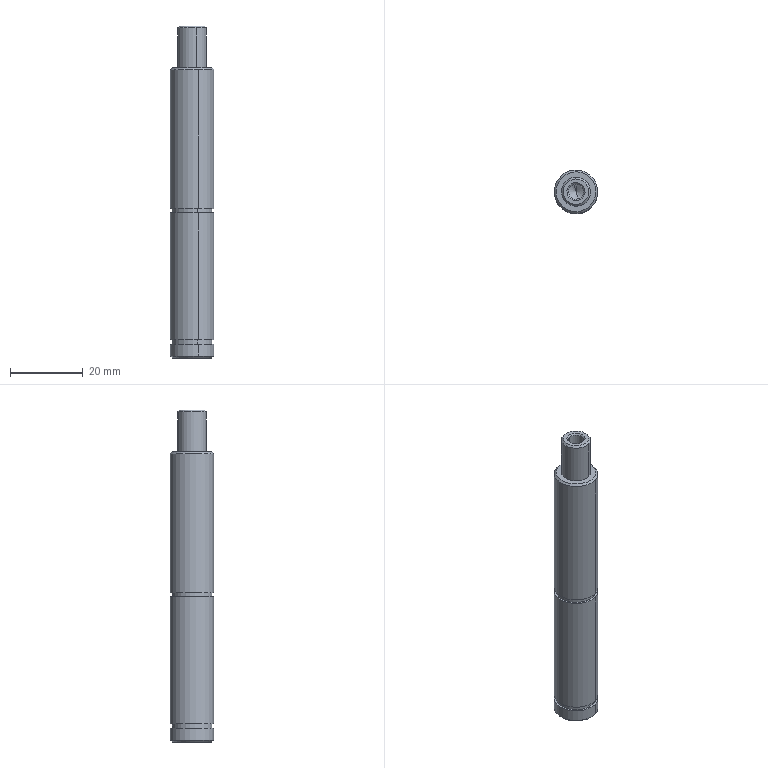Component | SolidWorks | GluePaperFeedingPressureRollerAssembly-1_YX-04-110GluePaperFeedingPressureRollerAxis-1 | 1 solid | 31 faces | box 12 x 12 x 91.5 mm | volume 9389 mm3 | cylinder 14 | cone 10 | plane 7 | commonest cylinder face diameters 12 x6 11 x4 8 x2 4.2 x2 | material Hard Chrome Rod
build123d program:
from build123d import *


with BuildPart() as part:
    # Sketch1 → Revolve1 (revolve)
    with BuildSketch(Plane.XY, mode=Mode.PRIVATE) as revolve1_sk:
        Polygon((12.6, 2.1), (13.862, 0), (91.5, 0), (91.5, 5.5), (91, 6), (87.7, 6), (87.7, 5.5), (86.5, 5.5), (86.5, 6), (51.5, 6), (51.5, 5.5), (50.3, 5.5), (50.3, 6), (12, 6), (11.5, 5.5), (11.5, 4), (0.5, 4), (0, 3.5), (0, 2.5), (0.4, 2.1), align=None)
    revolve(revolve1_sk.sketch.rotate(Axis((0, 0, 0), (1, 0, 0)), 270), axis=Axis((0, 0, 0), (1, 0, 0)))


solid = part.part

# Placed as in the assembly
solid = solid.moved(Location((-23.397, 0.262, 205.5), (0, 90, 0)))
STEP:
#1=CARTESIAN_POINT('',(-0.8978,-0.069,8.075));
#2=VERTEX_POINT('',#1);
#3=CARTESIAN_POINT('',(-0.9445,0.08963,8.075));
#4=VERTEX_POINT('',#3);
#5=CARTESIAN_POINT('',(-0.9212,0.01031,8.075));
#6=DIRECTION('',(-0.,0.,-1.));
#7=DIRECTION('',(-0.2824,0.9593,0.));
#8=AXIS2_PLACEMENT_3D('',#5,#6,#7);
#9=CIRCLE('',#8,0.08268);
#10=EDGE_CURVE('',#2,#4,#9,.T.);
#11=ORIENTED_EDGE('',*,*,#10,.T.);
#12=CARTESIAN_POINT('',(-0.9489,0.1047,8.091));
#13=VERTEX_POINT('',#12);
#14=CARTESIAN_POINT('',(-0.9489,0.1047,8.091));
#15=DIRECTION('',(-0.1997,0.6783,0.7071));
#16=VECTOR('',#15,39.37);
#17=LINE('',#14,#16);
#18=EDGE_CURVE('',#4,#13,#17,.T.);
#19=ORIENTED_EDGE('',*,*,#18,.T.);
#20=CARTESIAN_POINT('',(-0.8934,-0.0841,8.091));
#21=VERTEX_POINT('',#20);
#22=CARTESIAN_POINT('',(-0.9212,0.01031,8.091));
#23=DIRECTION('',(-0.,0.,-1.));
#24=DIRECTION('',(-0.2824,0.9593,0.));
#25=AXIS2_PLACEMENT_3D('',#22,#23,#24);
#26=CIRCLE('',#25,0.09843);
#27=EDGE_CURVE('',#21,#13,#26,.T.);
#28=ORIENTED_EDGE('',*,*,#27,.F.);
#29=CARTESIAN_POINT('',(-0.8934,-0.0841,8.091));
#30=DIRECTION('',(0.1997,-0.6783,0.7071));
#31=VECTOR('',#30,39.37);
#32=LINE('',#29,#31);
#33=EDGE_CURVE('',#2,#21,#32,.T.);
#34=ORIENTED_EDGE('',*,*,#33,.F.);
#35=EDGE_LOOP('',(#11,#19,#28,#34));
#36=FACE_OUTER_BOUND('',#35,.T.);
#37=CARTESIAN_POINT('',(-0.9212,0.01031,8.091));
#38=DIRECTION('',(0.,-0.,1.));
#39=DIRECTION('',(0.2824,-0.9593,0.));
#40=AXIS2_PLACEMENT_3D('',#37,#38,#39);
#41=CONICAL_SURFACE('',#40,0.09843,0.7854);
#42=ADVANCED_FACE('',(#36),#41,.F.);
#43=CARTESIAN_POINT('',(-0.9601,0.1425,8.091));
#44=VERTEX_POINT('',#43);
#45=CARTESIAN_POINT('',(-0.8822,-0.1219,8.091));
#46=VERTEX_POINT('',#45);
#47=CARTESIAN_POINT('',(-0.9212,0.01031,8.091));
#48=DIRECTION('',(-0.,0.,-1.));
#49=DIRECTION('',(-0.2824,0.9593,0.));
#50=AXIS2_PLACEMENT_3D('',#47,#48,#49);
#51=CIRCLE('',#50,0.1378);
#52=EDGE_CURVE('',#44,#46,#51,.T.);
#53=ORIENTED_EDGE('',*,*,#52,.T.);
#54=CARTESIAN_POINT('',(-0.8767,-0.1408,8.071));
#55=VERTEX_POINT('',#54);
#56=CARTESIAN_POINT('',(-0.8767,-0.1408,8.071));
#57=DIRECTION('',(0.1997,-0.6783,-0.7071));
#58=VECTOR('',#57,39.37);
#59=LINE('',#56,#58);
#60=EDGE_CURVE('',#46,#55,#59,.T.);
#61=ORIENTED_EDGE('',*,*,#60,.T.);
#62=CARTESIAN_POINT('',(-0.9656,0.1614,8.071));
#63=VERTEX_POINT('',#62);
#64=CARTESIAN_POINT('',(-0.9212,0.01031,8.071));
#65=DIRECTION('',(-0.,0.,-1.));
#66=DIRECTION('',(-0.2824,0.9593,0.));
#67=AXIS2_PLACEMENT_3D('',#64,#65,#66);
#68=CIRCLE('',#67,0.1575);
#69=EDGE_CURVE('',#63,#55,#68,.T.);
#70=ORIENTED_EDGE('',*,*,#69,.F.);
#71=CARTESIAN_POINT('',(-0.9656,0.1614,8.071));
#72=DIRECTION('',(-0.1997,0.6783,-0.7071));
#73=VECTOR('',#72,39.37);
#74=LINE('',#71,#73);
#75=EDGE_CURVE('',#44,#63,#74,.T.);
#76=ORIENTED_EDGE('',*,*,#75,.F.);
#77=EDGE_LOOP('',(#53,#61,#70,#76));
#78=FACE_OUTER_BOUND('',#77,.T.);
#79=CARTESIAN_POINT('',(-0.9212,0.01031,8.071));
#80=DIRECTION('',(-0.,0.,-1.));
#81=DIRECTION('',(-0.2824,0.9593,0.));
#82=AXIS2_PLACEMENT_3D('',#79,#80,#81);
#83=CONICAL_SURFACE('',#82,0.1575,0.7854);
#84=ADVANCED_FACE('',(#78),#83,.T.);
#85=ORIENTED_EDGE('',*,*,#69,.T.);
#86=CARTESIAN_POINT('',(-0.8767,-0.1408,7.638));
#87=VERTEX_POINT('',#86);
#88=CARTESIAN_POINT('',(-0.8767,-0.1408,8.091));
#89=DIRECTION('',(-0.,0.,-1.));
#90=VECTOR('',#89,39.37);
#91=LINE('',#88,#90);
#92=EDGE_CURVE('',#55,#87,#91,.T.);
#93=ORIENTED_EDGE('',*,*,#92,.T.);
#94=CARTESIAN_POINT('',(-0.9656,0.1614,7.638));
#95=VERTEX_POINT('',#94);
#96=CARTESIAN_POINT('',(-0.9212,0.01031,7.638));
#97=DIRECTION('',(-0.,0.,-1.));
#98=DIRECTION('',(-0.2824,0.9593,0.));
#99=AXIS2_PLACEMENT_3D('',#96,#97,#98);
#100=CIRCLE('',#99,0.1575);
#101=EDGE_CURVE('',#95,#87,#100,.T.);
#102=ORIENTED_EDGE('',*,*,#101,.F.);
#103=CARTESIAN_POINT('',(-0.9656,0.1614,8.091));
#104=DIRECTION('',(-0.,0.,-1.));
#105=VECTOR('',#104,39.37);
#106=LINE('',#103,#105);
#107=EDGE_CURVE('',#63,#95,#106,.T.);
#108=ORIENTED_EDGE('',*,*,#107,.F.);
#109=EDGE_LOOP('',(#85,#93,#102,#108));
#110=FACE_OUTER_BOUND('',#109,.T.);
#111=CARTESIAN_POINT('',(-0.9212,0.01031,8.091));
#112=DIRECTION('',(-0.,0.,-1.));
#113=DIRECTION('',(-0.2824,0.9593,0.));
#114=AXIS2_PLACEMENT_3D('',#111,#112,#113);
#115=CYLINDRICAL_SURFACE('',#114,0.1575);
#116=ADVANCED_FACE('',(#110),#115,.T.);
#117=CARTESIAN_POINT('',(-0.9823,0.218,7.638));
#118=VERTEX_POINT('',#117);
#119=CARTESIAN_POINT('',(-0.86,-0.1974,7.638));
#120=VERTEX_POINT('',#119);
#121=CARTESIAN_POINT('',(-0.9212,0.01031,7.638));
#122=DIRECTION('',(-0.,0.,-1.));
#123=DIRECTION('',(-0.2824,0.9593,0.));
#124=AXIS2_PLACEMENT_3D('',#121,#122,#123);
#125=CIRCLE('',#124,0.2165);
#126=EDGE_CURVE('',#118,#120,#125,.T.);
#127=ORIENTED_EDGE('',*,*,#126,.T.);
#128=CARTESIAN_POINT('',(-0.8544,-0.2163,7.618));
#129=VERTEX_POINT('',#128);
#130=CARTESIAN_POINT('',(-0.8544,-0.2163,7.618));
#131=DIRECTION('',(0.1997,-0.6783,-0.7071));
#132=VECTOR('',#131,39.37);
#133=LINE('',#130,#132);
#134=EDGE_CURVE('',#120,#129,#133,.T.);
#135=ORIENTED_EDGE('',*,*,#134,.T.);
#136=CARTESIAN_POINT('',(-0.9879,0.2369,7.618));
#137=VERTEX_POINT('',#136);
#138=CARTESIAN_POINT('',(-0.9212,0.01031,7.618));
#139=DIRECTION('',(-0.,0.,-1.));
#140=DIRECTION('',(-0.2824,0.9593,0.));
#141=AXIS2_PLACEMENT_3D('',#138,#139,#140);
#142=CIRCLE('',#141,0.2362);
#143=EDGE_CURVE('',#137,#129,#142,.T.);
#144=ORIENTED_EDGE('',*,*,#143,.F.);
#145=CARTESIAN_POINT('',(-0.9879,0.2369,7.618));
#146=DIRECTION('',(-0.1997,0.6783,-0.7071));
#147=VECTOR('',#146,39.37);
#148=LINE('',#145,#147);
#149=EDGE_CURVE('',#118,#137,#148,.T.);
#150=ORIENTED_EDGE('',*,*,#149,.F.);
#151=EDGE_LOOP('',(#127,#135,#144,#150));
#152=FACE_OUTER_BOUND('',#151,.T.);
#153=CARTESIAN_POINT('',(-0.9212,0.01031,7.618));
#154=DIRECTION('',(-0.,0.,-1.));
#155=DIRECTION('',(-0.2824,0.9593,0.));
#156=AXIS2_PLACEMENT_3D('',#153,#154,#155);
#157=CONICAL_SURFACE('',#156,0.2362,0.7854);
#158=ADVANCED_FACE('',(#152),#157,.T.);
#159=ORIENTED_EDGE('',*,*,#143,.T.);
#160=CARTESIAN_POINT('',(-0.8544,-0.2163,6.11));
#161=VERTEX_POINT('',#160);
#162=CARTESIAN_POINT('',(-0.8544,-0.2163,8.091));
#163=DIRECTION('',(-0.,0.,-1.));
#164=VECTOR('',#163,39.37);
#165=LINE('',#162,#164);
#166=EDGE_CURVE('',#129,#161,#165,.T.);
#167=ORIENTED_EDGE('',*,*,#166,.T.);
#168=CARTESIAN_POINT('',(-0.9879,0.2369,6.11));
#169=VERTEX_POINT('',#168);
#170=CARTESIAN_POINT('',(-0.9212,0.01031,6.11));
#171=DIRECTION('',(-0.,0.,-1.));
#172=DIRECTION('',(-0.2824,0.9593,0.));
#173=AXIS2_PLACEMENT_3D('',#170,#171,#172);
#174=CIRCLE('',#173,0.2362);
#175=EDGE_CURVE('',#169,#161,#174,.T.);
#176=ORIENTED_EDGE('',*,*,#175,.F.);
#177=CARTESIAN_POINT('',(-0.9879,0.2369,8.091));
#178=DIRECTION('',(-0.,0.,-1.));
#179=VECTOR('',#178,39.37);
#180=LINE('',#177,#179);
#181=EDGE_CURVE('',#137,#169,#180,.T.);
#182=ORIENTED_EDGE('',*,*,#181,.F.);
#183=EDGE_LOOP('',(#159,#167,#176,#182));
#184=FACE_OUTER_BOUND('',#183,.T.);
#185=CARTESIAN_POINT('',(-0.9212,0.01031,8.091));
#186=DIRECTION('',(-0.,0.,-1.));
#187=DIRECTION('',(-0.2824,0.9593,0.));
#188=AXIS2_PLACEMENT_3D('',#185,#186,#187);
#189=CYLINDRICAL_SURFACE('',#188,0.2362);
#190=ADVANCED_FACE('',(#184),#189,.T.);
#191=CARTESIAN_POINT('',(-0.9823,0.218,6.11));
#192=VERTEX_POINT('',#191);
#193=CARTESIAN_POINT('',(-0.86,-0.1974,6.11));
#194=VERTEX_POINT('',#193);
#195=CARTESIAN_POINT('',(-0.9212,0.01031,6.11));
#196=DIRECTION('',(-0.,0.,-1.));
#197=DIRECTION('',(-0.2824,0.9593,0.));
#198=AXIS2_PLACEMENT_3D('',#195,#196,#197);
#199=CIRCLE('',#198,0.2165);
#200=EDGE_CURVE('',#192,#194,#199,.T.);
#201=ORIENTED_EDGE('',*,*,#200,.T.);
#202=CARTESIAN_POINT('',(-0.86,-0.1974,6.063));
#203=VERTEX_POINT('',#202);
#204=CARTESIAN_POINT('',(-0.86,-0.1974,8.091));
#205=DIRECTION('',(-0.,0.,-1.));
#206=VECTOR('',#205,39.37);
#207=LINE('',#204,#206);
#208=EDGE_CURVE('',#194,#203,#207,.T.);
#209=ORIENTED_EDGE('',*,*,#208,.T.);
#210=CARTESIAN_POINT('',(-0.9823,0.218,6.063));
#211=VERTEX_POINT('',#210);
#212=CARTESIAN_POINT('',(-0.9212,0.01031,6.063));
#213=DIRECTION('',(-0.,0.,-1.));
#214=DIRECTION('',(-0.2824,0.9593,0.));
#215=AXIS2_PLACEMENT_3D('',#212,#213,#214);
#216=CIRCLE('',#215,0.2165);
#217=EDGE_CURVE('',#211,#203,#216,.T.);
#218=ORIENTED_EDGE('',*,*,#217,.F.);
#219=CARTESIAN_POINT('',(-0.9823,0.218,8.091));
#220=DIRECTION('',(-0.,0.,-1.));
#221=VECTOR('',#220,39.37);
#222=LINE('',#219,#221);
#223=EDGE_CURVE('',#192,#211,#222,.T.);
#224=ORIENTED_EDGE('',*,*,#223,.F.);
#225=EDGE_LOOP('',(#201,#209,#218,#224));
#226=FACE_OUTER_BOUND('',#225,.T.);
#227=CARTESIAN_POINT('',(-0.9212,0.01031,8.091));
#228=DIRECTION('',(-0.,0.,-1.));
#229=DIRECTION('',(-0.2824,0.9593,0.));
#230=AXIS2_PLACEMENT_3D('',#227,#228,#229);
#231=CYLINDRICAL_SURFACE('',#230,0.2165);
#232=ADVANCED_FACE('',(#226),#231,.T.);
#233=CARTESIAN_POINT('',(-0.9879,0.2369,6.063));
#234=VERTEX_POINT('',#233);
#235=CARTESIAN_POINT('',(-0.8544,-0.2163,6.063));
#236=VERTEX_POINT('',#235);
#237=CARTESIAN_POINT('',(-0.9212,0.01031,6.063));
#238=DIRECTION('',(-0.,0.,-1.));
#239=DIRECTION('',(-0.2824,0.9593,0.));
#240=AXIS2_PLACEMENT_3D('',#237,#238,#239);
#241=CIRCLE('',#240,0.2362);
#242=EDGE_CURVE('',#234,#236,#241,.T.);
#243=ORIENTED_EDGE('',*,*,#242,.T.);
#244=CARTESIAN_POINT('',(-0.8544,-0.2163,4.685));
#245=VERTEX_POINT('',#244);
#246=CARTESIAN_POINT('',(-0.8544,-0.2163,8.091));
#247=DIRECTION('',(-0.,0.,-1.));
#248=VECTOR('',#247,39.37);
#249=LINE('',#246,#248);
#250=EDGE_CURVE('',#236,#245,#249,.T.);
#251=ORIENTED_EDGE('',*,*,#250,.T.);
#252=CARTESIAN_POINT('',(-0.9879,0.2369,4.685));
#253=VERTEX_POINT('',#252);
#254=CARTESIAN_POINT('',(-0.9212,0.01031,4.685));
#255=DIRECTION('',(-0.,0.,-1.));
#256=DIRECTION('',(-0.2824,0.9593,0.));
#257=AXIS2_PLACEMENT_3D('',#254,#255,#256);
#258=CIRCLE('',#257,0.2362);
#259=EDGE_CURVE('',#253,#245,#258,.T.);
#260=ORIENTED_EDGE('',*,*,#259,.F.);
#261=CARTESIAN_POINT('',(-0.9879,0.2369,8.091));
#262=DIRECTION('',(-0.,0.,-1.));
#263=VECTOR('',#262,39.37);
#264=LINE('',#261,#263);
#265=EDGE_CURVE('',#234,#253,#264,.T.);
#266=ORIENTED_EDGE('',*,*,#265,.F.);
#267=EDGE_LOOP('',(#243,#251,#260,#266));
#268=FACE_OUTER_BOUND('',#267,.T.);
#269=CARTESIAN_POINT('',(-0.9212,0.01031,8.091));
#270=DIRECTION('',(-0.,0.,-1.));
#271=DIRECTION('',(-0.2824,0.9593,0.));
#272=AXIS2_PLACEMENT_3D('',#269,#270,#271);
#273=CYLINDRICAL_SURFACE('',#272,0.2362);
#274=ADVANCED_FACE('',(#268),#273,.T.);
#275=CARTESIAN_POINT('',(-0.9823,0.218,4.685));
#276=VERTEX_POINT('',#275);
#277=CARTESIAN_POINT('',(-0.86,-0.1974,4.685));
#278=VERTEX_POINT('',#277);
#279=CARTESIAN_POINT('',(-0.9212,0.01031,4.685));
#280=DIRECTION('',(-0.,0.,-1.));
#281=DIRECTION('',(-0.2824,0.9593,0.));
#282=AXIS2_PLACEMENT_3D('',#279,#280,#281);
#283=CIRCLE('',#282,0.2165);
#284=EDGE_CURVE('',#276,#278,#283,.T.);
#285=ORIENTED_EDGE('',*,*,#284,.T.);
#286=CARTESIAN_POINT('',(-0.86,-0.1974,4.638));
#287=VERTEX_POINT('',#286);
#288=CARTESIAN_POINT('',(-0.86,-0.1974,8.091));
#289=DIRECTION('',(-0.,0.,-1.));
#290=VECTOR('',#289,39.37);
#291=LINE('',#288,#290);
#292=EDGE_CURVE('',#278,#287,#291,.T.);
#293=ORIENTED_EDGE('',*,*,#292,.T.);
#294=CARTESIAN_POINT('',(-0.9823,0.218,4.638));
#295=VERTEX_POINT('',#294);
#296=CARTESIAN_POINT('',(-0.9212,0.01031,4.638));
#297=DIRECTION('',(-0.,0.,-1.));
#298=DIRECTION('',(-0.2824,0.9593,0.));
#299=AXIS2_PLACEMENT_3D('',#296,#297,#298);
#300=CIRCLE('',#299,0.2165);
#301=EDGE_CURVE('',#295,#287,#300,.T.);
#302=ORIENTED_EDGE('',*,*,#301,.F.);
#303=CARTESIAN_POINT('',(-0.9823,0.218,8.091));
#304=DIRECTION('',(-0.,0.,-1.));
#305=VECTOR('',#304,39.37);
#306=LINE('',#303,#305);
#307=EDGE_CURVE('',#276,#295,#306,.T.);
#308=ORIENTED_EDGE('',*,*,#307,.F.);
#309=EDGE_LOOP('',(#285,#293,#302,#308));
#310=FACE_OUTER_BOUND('',#309,.T.);
#311=CARTESIAN_POINT('',(-0.9212,0.01031,8.091));
#312=DIRECTION('',(-0.,0.,-1.));
#313=DIRECTION('',(-0.2824,0.9593,0.));
#314=AXIS2_PLACEMENT_3D('',#311,#312,#313);
#315=CYLINDRICAL_SURFACE('',#314,0.2165);
#316=ADVANCED_FACE('',(#310),#315,.T.);
#317=CARTESIAN_POINT('',(-0.9879,0.2369,4.638));
#318=VERTEX_POINT('',#317);
#319=CARTESIAN_POINT('',(-0.8544,-0.2163,4.638));
#320=VERTEX_POINT('',#319);
#321=CARTESIAN_POINT('',(-0.9212,0.01031,4.638));
#322=DIRECTION('',(-0.,0.,-1.));
#323=DIRECTION('',(-0.2824,0.9593,0.));
#324=AXIS2_PLACEMENT_3D('',#321,#322,#323);
#325=CIRCLE('',#324,0.2362);
#326=EDGE_CURVE('',#318,#320,#325,.T.);
#327=ORIENTED_EDGE('',*,*,#326,.T.);
#328=CARTESIAN_POINT('',(-0.8544,-0.2163,4.508));
#329=VERTEX_POINT('',#328);
#330=CARTESIAN_POINT('',(-0.8544,-0.2163,8.091));
#331=DIRECTION('',(-0.,0.,-1.));
#332=VECTOR('',#331,39.37);
#333=LINE('',#330,#332);
#334=EDGE_CURVE('',#320,#329,#333,.T.);
#335=ORIENTED_EDGE('',*,*,#334,.T.);
#336=CARTESIAN_POINT('',(-0.9879,0.2369,4.508));
#337=VERTEX_POINT('',#336);
#338=CARTESIAN_POINT('',(-0.9212,0.01031,4.508));
#339=DIRECTION('',(-0.,0.,-1.));
#340=DIRECTION('',(-0.2824,0.9593,0.));
#341=AXIS2_PLACEMENT_3D('',#338,#339,#340);
#342=CIRCLE('',#341,0.2362);
#343=EDGE_CURVE('',#337,#329,#342,.T.);
#344=ORIENTED_EDGE('',*,*,#343,.F.);
#345=CARTESIAN_POINT('',(-0.9879,0.2369,8.091));
#346=DIRECTION('',(-0.,0.,-1.));
#347=VECTOR('',#346,39.37);
#348=LINE('',#345,#347);
#349=EDGE_CURVE('',#318,#337,#348,.T.);
#350=ORIENTED_EDGE('',*,*,#349,.F.);
#351=EDGE_LOOP('',(#327,#335,#344,#350));
#352=FACE_OUTER_BOUND('',#351,.T.);
#353=CARTESIAN_POINT('',(-0.9212,0.01031,8.091));
#354=DIRECTION('',(-0.,0.,-1.));
#355=DIRECTION('',(-0.2824,0.9593,0.));
#356=AXIS2_PLACEMENT_3D('',#353,#354,#355);
#357=CYLINDRICAL_SURFACE('',#356,0.2362);
#358=ADVANCED_FACE('',(#352),#357,.T.);
#359=CARTESIAN_POINT('',(-0.9823,0.218,4.488));
#360=VERTEX_POINT('',#359);
#361=CARTESIAN_POINT('',(-0.86,-0.1974,4.488));
#362=VERTEX_POINT('',#361);
#363=CARTESIAN_POINT('',(-0.9212,0.01031,4.488));
#364=DIRECTION('',(-0.,0.,-1.));
#365=DIRECTION('',(-0.2824,0.9593,0.));
#366=AXIS2_PLACEMENT_3D('',#363,#364,#365);
#367=CIRCLE('',#366,0.2165);
#368=EDGE_CURVE('',#360,#362,#367,.T.);
#369=ORIENTED_EDGE('',*,*,#368,.F.);
#370=CARTESIAN_POINT('',(-0.9823,0.218,4.488));
#371=DIRECTION('',(-0.1997,0.6783,0.7071));
#372=VECTOR('',#371,39.37);
#373=LINE('',#370,#372);
#374=EDGE_CURVE('',#360,#337,#373,.T.);
#375=ORIENTED_EDGE('',*,*,#374,.T.);
#376=ORIENTED_EDGE('',*,*,#343,.T.);
#377=CARTESIAN_POINT('',(-0.86,-0.1974,4.488));
#378=DIRECTION('',(0.1997,-0.6783,0.7071));
#379=VECTOR('',#378,39.37);
#380=LINE('',#377,#379);
#381=EDGE_CURVE('',#362,#329,#380,.T.);
#382=ORIENTED_EDGE('',*,*,#381,.F.);
#383=EDGE_LOOP('',(#369,#375,#376,#382));
#384=FACE_OUTER_BOUND('',#383,.T.);
#385=CARTESIAN_POINT('',(-0.9212,0.01031,4.488));
#386=DIRECTION('',(0.,-0.,1.));
#387=DIRECTION('',(0.2824,-0.9593,0.));
#388=AXIS2_PLACEMENT_3D('',#385,#386,#387);
#389=CONICAL_SURFACE('',#388,0.2165,0.7854);
#390=ADVANCED_FACE('',(#384),#389,.T.);
#391=CARTESIAN_POINT('',(-0.9212,0.01031,7.545));
#392=VERTEX_POINT('',#391);
#393=CARTESIAN_POINT('',(-0.8978,-0.069,7.594));
#394=VERTEX_POINT('',#393);
#395=CARTESIAN_POINT('',(-0.8978,-0.069,7.594));
#396=DIRECTION('',(0.2421,-0.8223,0.515));
#397=VECTOR('',#396,39.37);
#398=LINE('',#395,#397);
#399=EDGE_CURVE('',#392,#394,#398,.T.);
#400=ORIENTED_EDGE('',*,*,#399,.F.);
#401=CARTESIAN_POINT('',(-0.9445,0.08963,7.594));
#402=VERTEX_POINT('',#401);
#403=CARTESIAN_POINT('',(-0.9445,0.08963,7.594));
#404=DIRECTION('',(-0.2421,0.8223,0.515));
#405=VECTOR('',#404,39.37);
#406=LINE('',#403,#405);
#407=EDGE_CURVE('',#392,#402,#406,.T.);
#408=ORIENTED_EDGE('',*,*,#407,.T.);
#409=CARTESIAN_POINT('',(-0.9212,0.01031,7.594));
#410=DIRECTION('',(-0.,0.,-1.));
#411=DIRECTION('',(-0.2824,0.9593,0.));
#412=AXIS2_PLACEMENT_3D('',#409,#410,#411);
#413=CIRCLE('',#412,0.08268);
#414=EDGE_CURVE('',#394,#402,#413,.T.);
#415=ORIENTED_EDGE('',*,*,#414,.F.);
#416=EDGE_LOOP('',(#400,#408,#415));
#417=FACE_OUTER_BOUND('',#416,.T.);
#418=CARTESIAN_POINT('',(-0.9212,0.01031,7.594));
#419=DIRECTION('',(0.,-0.,1.));
#420=DIRECTION('',(0.2824,-0.9593,0.));
#421=AXIS2_PLACEMENT_3D('',#418,#419,#420);
#422=CONICAL_SURFACE('',#421,0.08268,1.03);
#423=ADVANCED_FACE('',(#417),#422,.F.);
#424=ORIENTED_EDGE('',*,*,#10,.F.);
#425=CARTESIAN_POINT('',(-0.8978,-0.069,8.091));
#426=DIRECTION('',(-0.,0.,-1.));
#427=VECTOR('',#426,39.37);
#428=LINE('',#425,#427);
#429=EDGE_CURVE('',#2,#394,#428,.T.);
#430=ORIENTED_EDGE('',*,*,#429,.T.);
#431=ORIENTED_EDGE('',*,*,#414,.T.);
#432=CARTESIAN_POINT('',(-0.9445,0.08963,8.091));
#433=DIRECTION('',(-0.,0.,-1.));
#434=VECTOR('',#433,39.37);
#435=LINE('',#432,#434);
#436=EDGE_CURVE('',#4,#402,#435,.T.);
#437=ORIENTED_EDGE('',*,*,#436,.F.);
#438=EDGE_LOOP('',(#424,#430,#431,#437));
#439=FACE_OUTER_BOUND('',#438,.T.);
#440=CARTESIAN_POINT('',(-0.9212,0.01031,8.091));
#441=DIRECTION('',(-0.,0.,-1.));
#442=DIRECTION('',(-0.2824,0.9593,0.));
#443=AXIS2_PLACEMENT_3D('',#440,#441,#442);
#444=CYLINDRICAL_SURFACE('',#443,0.08268);
#445=ADVANCED_FACE('',(#439),#444,.F.);
#446=ORIENTED_EDGE('',*,*,#429,.F.);
#447=CARTESIAN_POINT('',(-0.9212,0.01031,8.075));
#448=DIRECTION('',(-0.,0.,-1.));
#449=DIRECTION('',(-0.2824,0.9593,0.));
#450=AXIS2_PLACEMENT_3D('',#447,#448,#449);
#451=CIRCLE('',#450,0.08268);
#452=EDGE_CURVE('',#4,#2,#451,.T.);
#453=ORIENTED_EDGE('',*,*,#452,.F.);
#454=ORIENTED_EDGE('',*,*,#436,.T.);
#455=CARTESIAN_POINT('',(-0.9212,0.01031,7.594));
#456=DIRECTION('',(-0.,0.,-1.));
#457=DIRECTION('',(-0.2824,0.9593,0.));
#458=AXIS2_PLACEMENT_3D('',#455,#456,#457);
#459=CIRCLE('',#458,0.08268);
#460=EDGE_CURVE('',#402,#394,#459,.T.);
#461=ORIENTED_EDGE('',*,*,#460,.T.);
#462=EDGE_LOOP('',(#446,#453,#454,#461));
#463=FACE_OUTER_BOUND('',#462,.T.);
#464=CARTESIAN_POINT('',(-0.9212,0.01031,8.091));
#465=DIRECTION('',(-0.,0.,-1.));
#466=DIRECTION('',(-0.2824,0.9593,0.));
#467=AXIS2_PLACEMENT_3D('',#464,#465,#466);
#468=CYLINDRICAL_SURFACE('',#467,0.08268);
#469=ADVANCED_FACE('',(#463),#468,.F.);
#470=ORIENTED_EDGE('',*,*,#407,.F.);
#471=ORIENTED_EDGE('',*,*,#399,.T.);
#472=ORIENTED_EDGE('',*,*,#460,.F.);
#473=EDGE_LOOP('',(#470,#471,#472));
#474=FACE_OUTER_BOUND('',#473,.T.);
#475=CARTESIAN_POINT('',(-0.9212,0.01031,7.594));
#476=DIRECTION('',(0.,-0.,1.));
#477=DIRECTION('',(0.2824,-0.9593,0.));
#478=AXIS2_PLACEMENT_3D('',#475,#476,#477);
#479=CONICAL_SURFACE('',#478,0.08268,1.03);
#480=ADVANCED_FACE('',(#474),#479,.F.);
#481=CARTESIAN_POINT('',(-0.9212,0.01031,4.488));
#482=DIRECTION('',(-0.,0.,-1.));
#483=DIRECTION('',(-0.2824,0.9593,0.));
#484=AXIS2_PLACEMENT_3D('',#481,#482,#483);
#485=CIRCLE('',#484,0.2165);
#486=EDGE_CURVE('',#362,#360,#485,.T.);
#487=ORIENTED_EDGE('',*,*,#486,.T.);
#488=ORIENTED_EDGE('',*,*,#368,.T.);
#489=EDGE_LOOP('',(#487,#488));
#490=FACE_OUTER_BOUND('',#489,.T.);
#491=CARTESIAN_POINT('',(-0.9212,0.01031,4.488));
#492=DIRECTION('',(-0.,0.,-1.));
#493=DIRECTION('',(-0.2824,0.9593,0.));
#494=AXIS2_PLACEMENT_3D('',#491,#492,#493);
#495=PLANE('',#494);
#496=ADVANCED_FACE('',(#490),#495,.T.);
#497=ORIENTED_EDGE('',*,*,#374,.F.);
#498=ORIENTED_EDGE('',*,*,#486,.F.);
#499=ORIENTED_EDGE('',*,*,#381,.T.);
#500=CARTESIAN_POINT('',(-0.9212,0.01031,4.508));
#501=DIRECTION('',(-0.,0.,-1.));
#502=DIRECTION('',(-0.2824,0.9593,0.));
#503=AXIS2_PLACEMENT_3D('',#500,#501,#502);
#504=CIRCLE('',#503,0.2362);
#505=EDGE_CURVE('',#329,#337,#504,.T.);
#506=ORIENTED_EDGE('',*,*,#505,.T.);
#507=EDGE_LOOP('',(#497,#498,#499,#506));
#508=FACE_OUTER_BOUND('',#507,.T.);
#509=CARTESIAN_POINT('',(-0.9212,0.01031,4.488));
#510=DIRECTION('',(0.,-0.,1.));
#511=DIRECTION('',(0.2824,-0.9593,0.));
#512=AXIS2_PLACEMENT_3D('',#509,#510,#511);
#513=CONICAL_SURFACE('',#512,0.2165,0.7854);
#514=ADVANCED_FACE('',(#508),#513,.T.);
#515=ORIENTED_EDGE('',*,*,#334,.F.);
#516=CARTESIAN_POINT('',(-0.9212,0.01031,4.638));
#517=DIRECTION('',(-0.,0.,-1.));
#518=DIRECTION('',(-0.2824,0.9593,0.));
#519=AXIS2_PLACEMENT_3D('',#516,#517,#518);
#520=CIRCLE('',#519,0.2362);
#521=EDGE_CURVE('',#320,#318,#520,.T.);
#522=ORIENTED_EDGE('',*,*,#521,.T.);
#523=ORIENTED_EDGE('',*,*,#349,.T.);
#524=ORIENTED_EDGE('',*,*,#505,.F.);
#525=EDGE_LOOP('',(#515,#522,#523,#524));
#526=FACE_OUTER_BOUND('',#525,.T.);
#527=CARTESIAN_POINT('',(-0.9212,0.01031,8.091));
#528=DIRECTION('',(-0.,0.,-1.));
#529=DIRECTION('',(-0.2824,0.9593,0.));
#530=AXIS2_PLACEMENT_3D('',#527,#528,#529);
#531=CYLINDRICAL_SURFACE('',#530,0.2362);
#532=ADVANCED_FACE('',(#526),#531,.T.);
#533=ORIENTED_EDGE('',*,*,#301,.T.);
#534=CARTESIAN_POINT('',(-0.9212,0.01031,4.638));
#535=DIRECTION('',(-0.,0.,-1.));
#536=DIRECTION('',(-0.2824,0.9593,0.));
#537=AXIS2_PLACEMENT_3D('',#534,#535,#536);
#538=CIRCLE('',#537,0.2165);
#539=EDGE_CURVE('',#287,#295,#538,.T.);
#540=ORIENTED_EDGE('',*,*,#539,.T.);
#541=EDGE_LOOP('',(#533,#540));
#542=FACE_BOUND('',#541,.T.);
#543=ORIENTED_EDGE('',*,*,#326,.F.);
#544=ORIENTED_EDGE('',*,*,#521,.F.);
#545=EDGE_LOOP('',(#543,#544));
#546=FACE_OUTER_BOUND('',#545,.T.);
#547=CARTESIAN_POINT('',(-0.6945,0.07702,4.638));
#548=DIRECTION('',(0.,-0.,1.));
#549=DIRECTION('',(0.2824,-0.9593,-0.));
#550=AXIS2_PLACEMENT_3D('',#547,#548,#549);
#551=PLANE('',#550);
#552=ADVANCED_FACE('',(#542,#546),#551,.T.);
#553=ORIENTED_EDGE('',*,*,#292,.F.);
#554=CARTESIAN_POINT('',(-0.9212,0.01031,4.685));
#555=DIRECTION('',(-0.,0.,-1.));
#556=DIRECTION('',(-0.2824,0.9593,0.));
#557=AXIS2_PLACEMENT_3D('',#554,#555,#556);
#558=CIRCLE('',#557,0.2165);
#559=EDGE_CURVE('',#278,#276,#558,.T.);
#560=ORIENTED_EDGE('',*,*,#559,.T.);
#561=ORIENTED_EDGE('',*,*,#307,.T.);
#562=ORIENTED_EDGE('',*,*,#539,.F.);
#563=EDGE_LOOP('',(#553,#560,#561,#562));
#564=FACE_OUTER_BOUND('',#563,.T.);
#565=CARTESIAN_POINT('',(-0.9212,0.01031,8.091));
#566=DIRECTION('',(-0.,0.,-1.));
#567=DIRECTION('',(-0.2824,0.9593,0.));
#568=AXIS2_PLACEMENT_3D('',#565,#566,#567);
#569=CYLINDRICAL_SURFACE('',#568,0.2165);
#570=ADVANCED_FACE('',(#564),#569,.T.);
#571=ORIENTED_EDGE('',*,*,#259,.T.);
#572=CARTESIAN_POINT('',(-0.9212,0.01031,4.685));
#573=DIRECTION('',(-0.,0.,-1.));
#574=DIRECTION('',(-0.2824,0.9593,0.));
#575=AXIS2_PLACEMENT_3D('',#572,#573,#574);
#576=CIRCLE('',#575,0.2362);
#577=EDGE_CURVE('',#245,#253,#576,.T.);
#578=ORIENTED_EDGE('',*,*,#577,.T.);
#579=EDGE_LOOP('',(#571,#578));
#580=FACE_OUTER_BOUND('',#579,.T.);
#581=ORIENTED_EDGE('',*,*,#284,.F.);
#582=ORIENTED_EDGE('',*,*,#559,.F.);
#583=EDGE_LOOP('',(#581,#582));
#584=FACE_BOUND('',#583,.T.);
#585=CARTESIAN_POINT('',(-0.7134,0.07146,4.685));
#586=DIRECTION('',(-0.,0.,-1.));
#587=DIRECTION('',(-0.2824,0.9593,0.));
#588=AXIS2_PLACEMENT_3D('',#585,#586,#587);
#589=PLANE('',#588);
#590=ADVANCED_FACE('',(#580,#584),#589,.T.);
#591=ORIENTED_EDGE('',*,*,#250,.F.);
#592=CARTESIAN_POINT('',(-0.9212,0.01031,6.063));
#593=DIRECTION('',(-0.,0.,-1.));
#594=DIRECTION('',(-0.2824,0.9593,0.));
#595=AXIS2_PLACEMENT_3D('',#592,#593,#594);
#596=CIRCLE('',#595,0.2362);
#597=EDGE_CURVE('',#236,#234,#596,.T.);
#598=ORIENTED_EDGE('',*,*,#597,.T.);
#599=ORIENTED_EDGE('',*,*,#265,.T.);
#600=ORIENTED_EDGE('',*,*,#577,.F.);
#601=EDGE_LOOP('',(#591,#598,#599,#600));
#602=FACE_OUTER_BOUND('',#601,.T.);
#603=CARTESIAN_POINT('',(-0.9212,0.01031,8.091));
#604=DIRECTION('',(-0.,0.,-1.));
#605=DIRECTION('',(-0.2824,0.9593,0.));
#606=AXIS2_PLACEMENT_3D('',#603,#604,#605);
#607=CYLINDRICAL_SURFACE('',#606,0.2362);
#608=ADVANCED_FACE('',(#602),#607,.T.);
#609=ORIENTED_EDGE('',*,*,#217,.T.);
#610=CARTESIAN_POINT('',(-0.9212,0.01031,6.063));
#611=DIRECTION('',(-0.,0.,-1.));
#612=DIRECTION('',(-0.2824,0.9593,0.));
#613=AXIS2_PLACEMENT_3D('',#610,#611,#612);
#614=CIRCLE('',#613,0.2165);
#615=EDGE_CURVE('',#203,#211,#614,.T.);
#616=ORIENTED_EDGE('',*,*,#615,.T.);
#617=EDGE_LOOP('',(#609,#616));
#618=FACE_BOUND('',#617,.T.);
#619=ORIENTED_EDGE('',*,*,#242,.F.);
#620=ORIENTED_EDGE('',*,*,#597,.F.);
#621=EDGE_LOOP('',(#619,#620));
#622=FACE_OUTER_BOUND('',#621,.T.);
#623=CARTESIAN_POINT('',(-0.6945,0.07702,6.063));
#624=DIRECTION('',(0.,-0.,1.));
#625=DIRECTION('',(0.2824,-0.9593,-0.));
#626=AXIS2_PLACEMENT_3D('',#623,#624,#625);
#627=PLANE('',#626);
#628=ADVANCED_FACE('',(#618,#622),#627,.T.);
#629=ORIENTED_EDGE('',*,*,#208,.F.);
#630=CARTESIAN_POINT('',(-0.9212,0.01031,6.11));
#631=DIRECTION('',(-0.,0.,-1.));
#632=DIRECTION('',(-0.2824,0.9593,0.));
#633=AXIS2_PLACEMENT_3D('',#630,#631,#632);
#634=CIRCLE('',#633,0.2165);
#635=EDGE_CURVE('',#194,#192,#634,.T.);
#636=ORIENTED_EDGE('',*,*,#635,.T.);
#637=ORIENTED_EDGE('',*,*,#223,.T.);
#638=ORIENTED_EDGE('',*,*,#615,.F.);
#639=EDGE_LOOP('',(#629,#636,#637,#638));
#640=FACE_OUTER_BOUND('',#639,.T.);
#641=CARTESIAN_POINT('',(-0.9212,0.01031,8.091));
#642=DIRECTION('',(-0.,0.,-1.));
#643=DIRECTION('',(-0.2824,0.9593,0.));
#644=AXIS2_PLACEMENT_3D('',#641,#642,#643);
#645=CYLINDRICAL_SURFACE('',#644,0.2165);
#646=ADVANCED_FACE('',(#640),#645,.T.);
#647=ORIENTED_EDGE('',*,*,#175,.T.);
#648=CARTESIAN_POINT('',(-0.9212,0.01031,6.11));
#649=DIRECTION('',(-0.,0.,-1.));
#650=DIRECTION('',(-0.2824,0.9593,0.));
#651=AXIS2_PLACEMENT_3D('',#648,#649,#650);
#652=CIRCLE('',#651,0.2362);
#653=EDGE_CURVE('',#161,#169,#652,.T.);
#654=ORIENTED_EDGE('',*,*,#653,.T.);
#655=EDGE_LOOP('',(#647,#654));
#656=FACE_OUTER_BOUND('',#655,.T.);
#657=ORIENTED_EDGE('',*,*,#200,.F.);
#658=ORIENTED_EDGE('',*,*,#635,.F.);
#659=EDGE_LOOP('',(#657,#658));
#660=FACE_BOUND('',#659,.T.);
#661=CARTESIAN_POINT('',(-0.7134,0.07146,6.11));
#662=DIRECTION('',(-0.,0.,-1.));
#663=DIRECTION('',(-0.2824,0.9593,0.));
#664=AXIS2_PLACEMENT_3D('',#661,#662,#663);
#665=PLANE('',#664);
#666=ADVANCED_FACE('',(#656,#660),#665,.T.);
#667=ORIENTED_EDGE('',*,*,#166,.F.);
#668=CARTESIAN_POINT('',(-0.9212,0.01031,7.618));
#669=DIRECTION('',(-0.,0.,-1.));
#670=DIRECTION('',(-0.2824,0.9593,0.));
#671=AXIS2_PLACEMENT_3D('',#668,#669,#670);
#672=CIRCLE('',#671,0.2362);
#673=EDGE_CURVE('',#129,#137,#672,.T.);
#674=ORIENTED_EDGE('',*,*,#673,.T.);
#675=ORIENTED_EDGE('',*,*,#181,.T.);
#676=ORIENTED_EDGE('',*,*,#653,.F.);
#677=EDGE_LOOP('',(#667,#674,#675,#676));
#678=FACE_OUTER_BOUND('',#677,.T.);
#679=CARTESIAN_POINT('',(-0.9212,0.01031,8.091));
#680=DIRECTION('',(-0.,0.,-1.));
#681=DIRECTION('',(-0.2824,0.9593,0.));
#682=AXIS2_PLACEMENT_3D('',#679,#680,#681);
#683=CYLINDRICAL_SURFACE('',#682,0.2362);
#684=ADVANCED_FACE('',(#678),#683,.T.);
#685=ORIENTED_EDGE('',*,*,#134,.F.);
#686=CARTESIAN_POINT('',(-0.9212,0.01031,7.638));
#687=DIRECTION('',(-0.,0.,-1.));
#688=DIRECTION('',(-0.2824,0.9593,0.));
#689=AXIS2_PLACEMENT_3D('',#686,#687,#688);
#690=CIRCLE('',#689,0.2165);
#691=EDGE_CURVE('',#120,#118,#690,.T.);
#692=ORIENTED_EDGE('',*,*,#691,.T.);
#693=ORIENTED_EDGE('',*,*,#149,.T.);
#694=ORIENTED_EDGE('',*,*,#673,.F.);
#695=EDGE_LOOP('',(#685,#692,#693,#694));
#696=FACE_OUTER_BOUND('',#695,.T.);
#697=CARTESIAN_POINT('',(-0.9212,0.01031,7.618));
#698=DIRECTION('',(-0.,0.,-1.));
#699=DIRECTION('',(-0.2824,0.9593,0.));
#700=AXIS2_PLACEMENT_3D('',#697,#698,#699);
#701=CONICAL_SURFACE('',#700,0.2362,0.7854);
#702=ADVANCED_FACE('',(#696),#701,.T.);
#703=ORIENTED_EDGE('',*,*,#101,.T.);
#704=CARTESIAN_POINT('',(-0.9212,0.01031,7.638));
#705=DIRECTION('',(-0.,0.,-1.));
#706=DIRECTION('',(-0.2824,0.9593,0.));
#707=AXIS2_PLACEMENT_3D('',#704,#705,#706);
#708=CIRCLE('',#707,0.1575);
#709=EDGE_CURVE('',#87,#95,#708,.T.);
#710=ORIENTED_EDGE('',*,*,#709,.T.);
#711=EDGE_LOOP('',(#703,#710));
#712=FACE_BOUND('',#711,.T.);
#713=ORIENTED_EDGE('',*,*,#126,.F.);
#714=ORIENTED_EDGE('',*,*,#691,.F.);
#715=EDGE_LOOP('',(#713,#714));
#716=FACE_OUTER_BOUND('',#715,.T.);
#717=CARTESIAN_POINT('',(-0.7134,0.07146,7.638));
#718=DIRECTION('',(0.,-0.,1.));
#719=DIRECTION('',(0.2824,-0.9593,-0.));
#720=AXIS2_PLACEMENT_3D('',#717,#718,#719);
#721=PLANE('',#720);
#722=ADVANCED_FACE('',(#712,#716),#721,.T.);
#723=ORIENTED_EDGE('',*,*,#92,.F.);
#724=CARTESIAN_POINT('',(-0.9212,0.01031,8.071));
#725=DIRECTION('',(-0.,0.,-1.));
#726=DIRECTION('',(-0.2824,0.9593,0.));
#727=AXIS2_PLACEMENT_3D('',#724,#725,#726);
#728=CIRCLE('',#727,0.1575);
#729=EDGE_CURVE('',#55,#63,#728,.T.);
#730=ORIENTED_EDGE('',*,*,#729,.T.);
#731=ORIENTED_EDGE('',*,*,#107,.T.);
#732=ORIENTED_EDGE('',*,*,#709,.F.);
#733=EDGE_LOOP('',(#723,#730,#731,#732));
#734=FACE_OUTER_BOUND('',#733,.T.);
#735=CARTESIAN_POINT('',(-0.9212,0.01031,8.091));
#736=DIRECTION('',(-0.,0.,-1.));
#737=DIRECTION('',(-0.2824,0.9593,0.));
#738=AXIS2_PLACEMENT_3D('',#735,#736,#737);
#739=CYLINDRICAL_SURFACE('',#738,0.1575);
#740=ADVANCED_FACE('',(#734),#739,.T.);
#741=ORIENTED_EDGE('',*,*,#60,.F.);
#742=CARTESIAN_POINT('',(-0.9212,0.01031,8.091));
#743=DIRECTION('',(-0.,0.,-1.));
#744=DIRECTION('',(-0.2824,0.9593,0.));
#745=AXIS2_PLACEMENT_3D('',#742,#743,#744);
#746=CIRCLE('',#745,0.1378);
#747=EDGE_CURVE('',#46,#44,#746,.T.);
#748=ORIENTED_EDGE('',*,*,#747,.T.);
#749=ORIENTED_EDGE('',*,*,#75,.T.);
#750=ORIENTED_EDGE('',*,*,#729,.F.);
#751=EDGE_LOOP('',(#741,#748,#749,#750));
#752=FACE_OUTER_BOUND('',#751,.T.);
#753=CARTESIAN_POINT('',(-0.9212,0.01031,8.071));
#754=DIRECTION('',(-0.,0.,-1.));
#755=DIRECTION('',(-0.2824,0.9593,0.));
#756=AXIS2_PLACEMENT_3D('',#753,#754,#755);
#757=CONICAL_SURFACE('',#756,0.1575,0.7854);
#758=ADVANCED_FACE('',(#752),#757,.T.);
#759=ORIENTED_EDGE('',*,*,#27,.T.);
#760=CARTESIAN_POINT('',(-0.9212,0.01031,8.091));
#761=DIRECTION('',(-0.,0.,-1.));
#762=DIRECTION('',(-0.2824,0.9593,0.));
#763=AXIS2_PLACEMENT_3D('',#760,#761,#762);
#764=CIRCLE('',#763,0.09843);
#765=EDGE_CURVE('',#13,#21,#764,.T.);
#766=ORIENTED_EDGE('',*,*,#765,.T.);
#767=EDGE_LOOP('',(#759,#766));
#768=FACE_BOUND('',#767,.T.);
#769=ORIENTED_EDGE('',*,*,#52,.F.);
#770=ORIENTED_EDGE('',*,*,#747,.F.);
#771=EDGE_LOOP('',(#769,#770));
#772=FACE_OUTER_BOUND('',#771,.T.);
#773=CARTESIAN_POINT('',(-0.789,0.04923,8.091));
#774=DIRECTION('',(0.,-0.,1.));
#775=DIRECTION('',(0.2824,-0.9593,-0.));
#776=AXIS2_PLACEMENT_3D('',#773,#774,#775);
#777=PLANE('',#776);
#778=ADVANCED_FACE('',(#768,#772),#777,.T.);
#779=ORIENTED_EDGE('',*,*,#18,.F.);
#780=ORIENTED_EDGE('',*,*,#452,.T.);
#781=ORIENTED_EDGE('',*,*,#33,.T.);
#782=ORIENTED_EDGE('',*,*,#765,.F.);
#783=EDGE_LOOP('',(#779,#780,#781,#782));
#784=FACE_OUTER_BOUND('',#783,.T.);
#785=CARTESIAN_POINT('',(-0.9212,0.01031,8.091));
#786=DIRECTION('',(0.,-0.,1.));
#787=DIRECTION('',(0.2824,-0.9593,0.));
#788=AXIS2_PLACEMENT_3D('',#785,#786,#787);
#789=CONICAL_SURFACE('',#788,0.09843,0.7854);
#790=ADVANCED_FACE('',(#784),#789,.F.);
#791=CLOSED_SHELL('',(#42,#84,#116,#158,#190,#232,#274,#316,#358,#390,#423,#445,#469,#480,#496,#514,#532,#552,#570,#590,#608,#628,#646,#666,#684,#702,#722,#740,#758,#778,#790));
#792=MANIFOLD_SOLID_BREP('',#791);
#793=CARTESIAN_POINT('',(0.,0.,0.));
#794=DIRECTION('',(0.,0.,1.));
#795=DIRECTION('',(1.,0.,0.));
#796=AXIS2_PLACEMENT_3D('',#793,#794,#795);
#797=(LENGTH_UNIT()NAMED_UNIT(*)SI_UNIT($,.METRE.));
#798=LENGTH_MEASURE_WITH_UNIT(LENGTH_MEASURE(0.0254),#797);
#799=DIMENSIONAL_EXPONENTS(1.,0.,0.,0.,0.,0.,0.);
#800=(CONVERSION_BASED_UNIT('',#798)LENGTH_UNIT()NAMED_UNIT(#799));
#801=UNCERTAINTY_MEASURE_WITH_UNIT(LENGTH_MEASURE(0.00001),#800,'','');
#802=(NAMED_UNIT(*)PLANE_ANGLE_UNIT()SI_UNIT($,.RADIAN.));
#803=(NAMED_UNIT(*)SI_UNIT($,.STERADIAN.)SOLID_ANGLE_UNIT());
#804=(GEOMETRIC_REPRESENTATION_CONTEXT(3)GLOBAL_UNCERTAINTY_ASSIGNED_CONTEXT((#801))GLOBAL_UNIT_ASSIGNED_CONTEXT((#800,#802,#803))REPRESENTATION_CONTEXT('',''));
#805=ADVANCED_BREP_SHAPE_REPRESENTATION('',(#792,#796),#804);
#806=COLOUR_RGB('',0.7922,0.8196,0.9333);
#807=FILL_AREA_STYLE_COLOUR('',#806);
#808=FILL_AREA_STYLE('',(#807));
#809=SURFACE_STYLE_FILL_AREA(#808);
#810=SURFACE_SIDE_STYLE('',(#809));
#811=SURFACE_STYLE_USAGE(.BOTH.,#810);
#812=PRESENTATION_STYLE_ASSIGNMENT((#811));
#813=STYLED_ITEM('',(#812),#792);
#814=PRESENTATION_LAYER_ASSIGNMENT('','',(#813));
#815=(LENGTH_UNIT()NAMED_UNIT(*)SI_UNIT($,.METRE.));
#816=LENGTH_MEASURE_WITH_UNIT(LENGTH_MEASURE(0.0254),#815);
#817=DIMENSIONAL_EXPONENTS(1.,0.,0.,0.,0.,0.,0.);
#818=(CONVERSION_BASED_UNIT('',#816)LENGTH_UNIT()NAMED_UNIT(#817));
#819=UNCERTAINTY_MEASURE_WITH_UNIT(LENGTH_MEASURE(0.00001),#818,'','');
#820=(NAMED_UNIT(*)PLANE_ANGLE_UNIT()SI_UNIT($,.RADIAN.));
#821=(NAMED_UNIT(*)SI_UNIT($,.STERADIAN.)SOLID_ANGLE_UNIT());
#822=(GEOMETRIC_REPRESENTATION_CONTEXT(3)GLOBAL_UNCERTAINTY_ASSIGNED_CONTEXT((#819))GLOBAL_UNIT_ASSIGNED_CONTEXT((#818,#820,#821))REPRESENTATION_CONTEXT('',''));
#823=MECHANICAL_DESIGN_GEOMETRIC_PRESENTATION_REPRESENTATION('',(#813),#822);